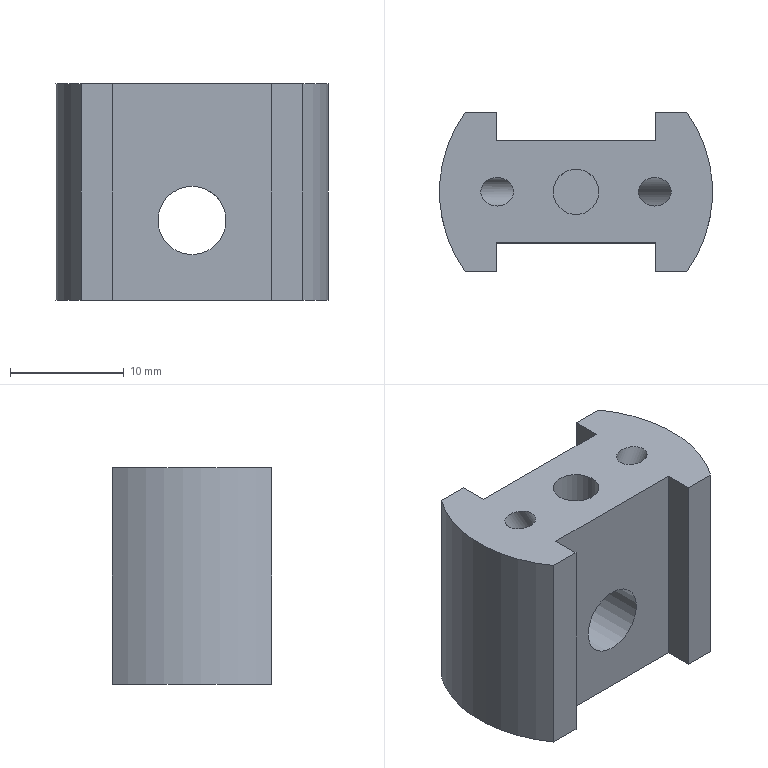Component | NX | PISTON_CONN_BLOCK | 1 solid | 19 faces | volume 4234 mm3 | plane 13 | cylinder 6 | commonest cylinder face diameters 24 x2 2.5 x2 6 x1 4 x1